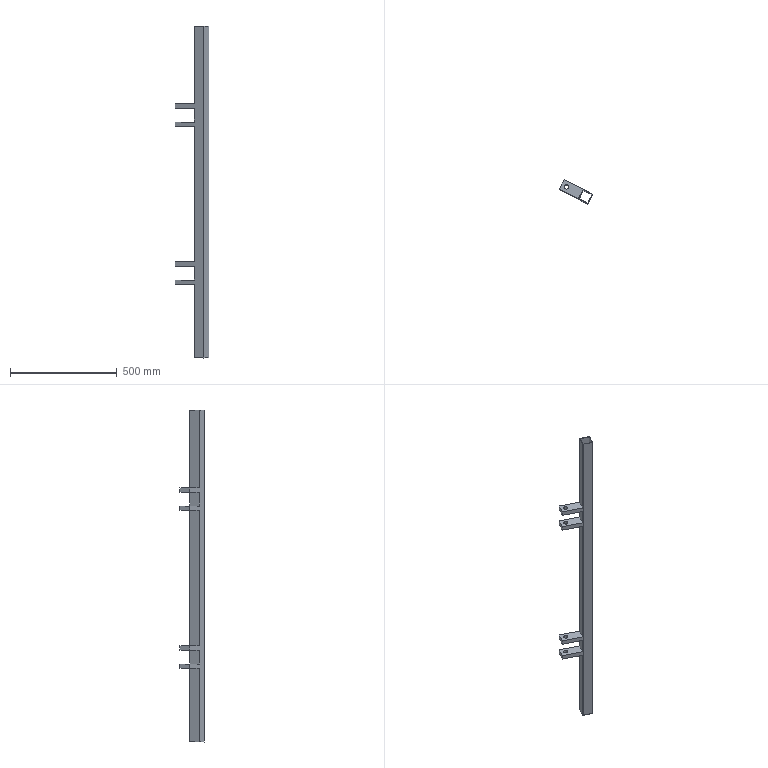Component | SolidWorks | Part13-1 | 1 solid | 34 faces | box 156.4 x 112.41 x 1554 mm | volume 971603 mm3 | plane 26 | cylinder 8 | commonest cylinder face diameters 20 x8
build123d program:
from build123d import *

# Parameters (mm, degrees)
SKETCH1_W           = 1554
SKETCH1_H           = 50
BOSS_EXTRUDE2_DEPTH = 50
SHELL1_T            = -2
SKETCH2_W           = 20
SKETCH2_H           = 100
BOSS_EXTRUDE3_DEPTH = 50
SKETCH3_R           = 10
CUT_EXTRUDE1_DEPTH  = 1195.898


with BuildPart() as part:
    # Sketch1 → Boss-Extrude2 (new body)
    with BuildSketch(Plane.XY):
        with Locations((715.859, 38.721)):
            Rectangle(SKETCH1_W, SKETCH1_H)
    extrude(amount=BOSS_EXTRUDE2_DEPTH)

    # Shell1
    shell1_openings = [part.faces().sort_by_distance(p)[0] for p in [
        (1492.859, 38.721, 25),
        (-61.141, 38.721, 25),
    ]]
    offset(amount=SHELL1_T, openings=shell1_openings, kind=Kind.INTERSECTION)

    # Sketch2 → Boss-Extrude3 (add)
    with BuildSketch(Plane.XZ.offset(-13.721)):
        with Locations((398.859, -50)):
            Rectangle(SKETCH2_W, SKETCH2_H)
        with Locations((313.859, -50)):
            Rectangle(SKETCH2_W, SKETCH2_H)
        with Locations((1052.859, -50)):
            Rectangle(SKETCH2_W, SKETCH2_H)
        with Locations((1137.859, -50)):
            Rectangle(SKETCH2_W, SKETCH2_H)
    extrude(amount=-BOSS_EXTRUDE3_DEPTH)

    # Sketch3 → Cut-Extrude1 (cut, through all)
    with BuildSketch(Plane.ZY.offset(-303.859)):
        with Locations((-75, 38.721)):
            Circle(SKETCH3_R)
    extrude(amount=-CUT_EXTRUDE1_DEPTH, mode=Mode.SUBTRACT)


solid = part.part

# Placed as in the assembly
solid = solid.moved(Location((-204.696, -928.158, 2528.83), (90, 63.121, -90)))
STEP:
#1=COLOUR_RGB('',0.7922,0.8196,0.9333);
#2=FILL_AREA_STYLE_COLOUR('',#1);
#3=FILL_AREA_STYLE('',(#2));
#4=SURFACE_STYLE_FILL_AREA(#3);
#5=SURFACE_SIDE_STYLE('',(#4));
#6=SURFACE_STYLE_USAGE(.BOTH.,#5);
#7=PRESENTATION_STYLE_ASSIGNMENT((#6));
#8=CARTESIAN_POINT('',(-9.652,-34.025,83.463));
#9=VERTEX_POINT('',#8);
#10=CARTESIAN_POINT('',(-10.355,-33.669,83.463));
#11=VERTEX_POINT('',#10);
#12=CARTESIAN_POINT('',(-10.003,-33.847,83.463));
#13=DIRECTION('',(0.,0.,-1.));
#14=DIRECTION('',(-0.892,0.4521,0.));
#15=AXIS2_PLACEMENT_3D('',#12,#13,#14);
#16=CIRCLE('',#15,0.3937);
#17=EDGE_CURVE('',#9,#11,#16,.T.);
#18=ORIENTED_EDGE('',*,*,#17,.T.);
#19=CARTESIAN_POINT('',(-10.355,-33.669,84.251));
#20=VERTEX_POINT('',#19);
#21=CARTESIAN_POINT('',(-10.355,-33.669,40.786));
#22=DIRECTION('',(-0.,-0.,1.));
#23=VECTOR('',#22,39.37);
#24=LINE('',#21,#23);
#25=EDGE_CURVE('',#11,#20,#24,.T.);
#26=ORIENTED_EDGE('',*,*,#25,.T.);
#27=CARTESIAN_POINT('',(-9.652,-34.025,84.251));
#28=VERTEX_POINT('',#27);
#29=CARTESIAN_POINT('',(-10.003,-33.847,84.251));
#30=DIRECTION('',(-0.,-0.,1.));
#31=DIRECTION('',(0.892,-0.4521,-0.));
#32=AXIS2_PLACEMENT_3D('',#29,#30,#31);
#33=CIRCLE('',#32,0.3937);
#34=EDGE_CURVE('',#20,#28,#33,.T.);
#35=ORIENTED_EDGE('',*,*,#34,.T.);
#36=CARTESIAN_POINT('',(-9.652,-34.025,40.786));
#37=DIRECTION('',(-0.,-0.,1.));
#38=VECTOR('',#37,39.37);
#39=LINE('',#36,#38);
#40=EDGE_CURVE('',#9,#28,#39,.T.);
#41=ORIENTED_EDGE('',*,*,#40,.F.);
#42=EDGE_LOOP('',(#18,#26,#35,#41));
#43=FACE_OUTER_BOUND('',#42,.T.);
#44=CARTESIAN_POINT('',(-10.003,-33.847,40.786));
#45=DIRECTION('',(-0.,-0.,1.));
#46=DIRECTION('',(0.892,-0.4521,-0.));
#47=AXIS2_PLACEMENT_3D('',#44,#45,#46);
#48=CYLINDRICAL_SURFACE('',#47,0.3937);
#49=ADVANCED_FACE('',(#43),#48,.F.);
#50=CARTESIAN_POINT('',(-9.652,-34.025,86.81));
#51=VERTEX_POINT('',#50);
#52=CARTESIAN_POINT('',(-10.355,-33.669,86.81));
#53=VERTEX_POINT('',#52);
#54=CARTESIAN_POINT('',(-10.003,-33.847,86.81));
#55=DIRECTION('',(0.,0.,-1.));
#56=DIRECTION('',(-0.892,0.4521,0.));
#57=AXIS2_PLACEMENT_3D('',#54,#55,#56);
#58=CIRCLE('',#57,0.3937);
#59=EDGE_CURVE('',#51,#53,#58,.T.);
#60=ORIENTED_EDGE('',*,*,#59,.T.);
#61=CARTESIAN_POINT('',(-10.355,-33.669,87.597));
#62=VERTEX_POINT('',#61);
#63=CARTESIAN_POINT('',(-10.355,-33.669,40.786));
#64=DIRECTION('',(-0.,-0.,1.));
#65=VECTOR('',#64,39.37);
#66=LINE('',#63,#65);
#67=EDGE_CURVE('',#53,#62,#66,.T.);
#68=ORIENTED_EDGE('',*,*,#67,.T.);
#69=CARTESIAN_POINT('',(-9.652,-34.025,87.597));
#70=VERTEX_POINT('',#69);
#71=CARTESIAN_POINT('',(-10.003,-33.847,87.597));
#72=DIRECTION('',(-0.,-0.,1.));
#73=DIRECTION('',(0.892,-0.4521,-0.));
#74=AXIS2_PLACEMENT_3D('',#71,#72,#73);
#75=CIRCLE('',#74,0.3937);
#76=EDGE_CURVE('',#62,#70,#75,.T.);
#77=ORIENTED_EDGE('',*,*,#76,.T.);
#78=CARTESIAN_POINT('',(-9.652,-34.025,40.786));
#79=DIRECTION('',(-0.,-0.,1.));
#80=VECTOR('',#79,39.37);
#81=LINE('',#78,#80);
#82=EDGE_CURVE('',#51,#70,#81,.T.);
#83=ORIENTED_EDGE('',*,*,#82,.F.);
#84=EDGE_LOOP('',(#60,#68,#77,#83));
#85=FACE_OUTER_BOUND('',#84,.T.);
#86=CARTESIAN_POINT('',(-10.003,-33.847,40.786));
#87=DIRECTION('',(-0.,-0.,1.));
#88=DIRECTION('',(0.892,-0.4521,-0.));
#89=AXIS2_PLACEMENT_3D('',#86,#87,#88);
#90=CYLINDRICAL_SURFACE('',#89,0.3937);
#91=ADVANCED_FACE('',(#85),#90,.F.);
#92=CARTESIAN_POINT('',(-9.652,-34.025,57.715));
#93=VERTEX_POINT('',#92);
#94=CARTESIAN_POINT('',(-10.355,-33.669,57.715));
#95=VERTEX_POINT('',#94);
#96=CARTESIAN_POINT('',(-10.003,-33.847,57.715));
#97=DIRECTION('',(0.,0.,-1.));
#98=DIRECTION('',(-0.892,0.4521,0.));
#99=AXIS2_PLACEMENT_3D('',#96,#97,#98);
#100=CIRCLE('',#99,0.3937);
#101=EDGE_CURVE('',#93,#95,#100,.T.);
#102=ORIENTED_EDGE('',*,*,#101,.T.);
#103=CARTESIAN_POINT('',(-10.355,-33.669,58.503));
#104=VERTEX_POINT('',#103);
#105=CARTESIAN_POINT('',(-10.355,-33.669,40.786));
#106=DIRECTION('',(-0.,-0.,1.));
#107=VECTOR('',#106,39.37);
#108=LINE('',#105,#107);
#109=EDGE_CURVE('',#95,#104,#108,.T.);
#110=ORIENTED_EDGE('',*,*,#109,.T.);
#111=CARTESIAN_POINT('',(-9.652,-34.025,58.503));
#112=VERTEX_POINT('',#111);
#113=CARTESIAN_POINT('',(-10.003,-33.847,58.503));
#114=DIRECTION('',(-0.,-0.,1.));
#115=DIRECTION('',(0.892,-0.4521,-0.));
#116=AXIS2_PLACEMENT_3D('',#113,#114,#115);
#117=CIRCLE('',#116,0.3937);
#118=EDGE_CURVE('',#104,#112,#117,.T.);
#119=ORIENTED_EDGE('',*,*,#118,.T.);
#120=CARTESIAN_POINT('',(-9.652,-34.025,40.786));
#121=DIRECTION('',(-0.,-0.,1.));
#122=VECTOR('',#121,39.37);
#123=LINE('',#120,#122);
#124=EDGE_CURVE('',#93,#112,#123,.T.);
#125=ORIENTED_EDGE('',*,*,#124,.F.);
#126=EDGE_LOOP('',(#102,#110,#119,#125));
#127=FACE_OUTER_BOUND('',#126,.T.);
#128=CARTESIAN_POINT('',(-10.003,-33.847,40.786));
#129=DIRECTION('',(-0.,-0.,1.));
#130=DIRECTION('',(0.892,-0.4521,-0.));
#131=AXIS2_PLACEMENT_3D('',#128,#129,#130);
#132=CYLINDRICAL_SURFACE('',#131,0.3937);
#133=ADVANCED_FACE('',(#127),#132,.F.);
#134=CARTESIAN_POINT('',(-9.652,-34.025,54.369));
#135=VERTEX_POINT('',#134);
#136=CARTESIAN_POINT('',(-10.355,-33.669,54.369));
#137=VERTEX_POINT('',#136);
#138=CARTESIAN_POINT('',(-10.003,-33.847,54.369));
#139=DIRECTION('',(0.,0.,-1.));
#140=DIRECTION('',(-0.892,0.4521,0.));
#141=AXIS2_PLACEMENT_3D('',#138,#139,#140);
#142=CIRCLE('',#141,0.3937);
#143=EDGE_CURVE('',#135,#137,#142,.T.);
#144=ORIENTED_EDGE('',*,*,#143,.T.);
#145=CARTESIAN_POINT('',(-10.355,-33.669,55.156));
#146=VERTEX_POINT('',#145);
#147=CARTESIAN_POINT('',(-10.355,-33.669,40.786));
#148=DIRECTION('',(-0.,-0.,1.));
#149=VECTOR('',#148,39.37);
#150=LINE('',#147,#149);
#151=EDGE_CURVE('',#137,#146,#150,.T.);
#152=ORIENTED_EDGE('',*,*,#151,.T.);
#153=CARTESIAN_POINT('',(-9.652,-34.025,55.156));
#154=VERTEX_POINT('',#153);
#155=CARTESIAN_POINT('',(-10.003,-33.847,55.156));
#156=DIRECTION('',(-0.,-0.,1.));
#157=DIRECTION('',(0.892,-0.4521,-0.));
#158=AXIS2_PLACEMENT_3D('',#155,#156,#157);
#159=CIRCLE('',#158,0.3937);
#160=EDGE_CURVE('',#146,#154,#159,.T.);
#161=ORIENTED_EDGE('',*,*,#160,.T.);
#162=CARTESIAN_POINT('',(-9.652,-34.025,40.786));
#163=DIRECTION('',(-0.,-0.,1.));
#164=VECTOR('',#163,39.37);
#165=LINE('',#162,#164);
#166=EDGE_CURVE('',#135,#154,#165,.T.);
#167=ORIENTED_EDGE('',*,*,#166,.F.);
#168=EDGE_LOOP('',(#144,#152,#161,#167));
#169=FACE_OUTER_BOUND('',#168,.T.);
#170=CARTESIAN_POINT('',(-10.003,-33.847,40.786));
#171=DIRECTION('',(-0.,-0.,1.));
#172=DIRECTION('',(0.892,-0.4521,-0.));
#173=AXIS2_PLACEMENT_3D('',#170,#171,#172);
#174=CYLINDRICAL_SURFACE('',#173,0.3937);
#175=ADVANCED_FACE('',(#169),#174,.F.);
#176=CARTESIAN_POINT('',(-6.925,-34.304,54.369));
#177=VERTEX_POINT('',#176);
#178=CARTESIAN_POINT('',(-7.815,-36.06,54.369));
#179=VERTEX_POINT('',#178);
#180=CARTESIAN_POINT('',(-6.925,-34.304,54.369));
#181=DIRECTION('',(-0.4521,-0.892,-0.));
#182=VECTOR('',#181,39.37);
#183=LINE('',#180,#182);
#184=EDGE_CURVE('',#177,#179,#183,.T.);
#185=ORIENTED_EDGE('',*,*,#184,.F.);
#186=CARTESIAN_POINT('',(-6.925,-34.304,40.786));
#187=VERTEX_POINT('',#186);
#188=CARTESIAN_POINT('',(-6.925,-34.304,101.967));
#189=DIRECTION('',(-0.,-0.,1.));
#190=VECTOR('',#189,39.37);
#191=LINE('',#188,#190);
#192=EDGE_CURVE('',#187,#177,#191,.T.);
#193=ORIENTED_EDGE('',*,*,#192,.F.);
#194=CARTESIAN_POINT('',(-7.815,-36.06,40.786));
#195=VERTEX_POINT('',#194);
#196=CARTESIAN_POINT('',(-6.925,-34.304,40.786));
#197=DIRECTION('',(0.4521,0.892,0.));
#198=VECTOR('',#197,39.37);
#199=LINE('',#196,#198);
#200=EDGE_CURVE('',#195,#187,#199,.T.);
#201=ORIENTED_EDGE('',*,*,#200,.F.);
#202=CARTESIAN_POINT('',(-7.815,-36.06,101.967));
#203=DIRECTION('',(0.,0.,-1.));
#204=VECTOR('',#203,39.37);
#205=LINE('',#202,#204);
#206=EDGE_CURVE('',#179,#195,#205,.T.);
#207=ORIENTED_EDGE('',*,*,#206,.F.);
#208=EDGE_LOOP('',(#185,#193,#201,#207));
#209=FACE_OUTER_BOUND('',#208,.T.);
#210=CARTESIAN_POINT('',(-8.059,-36.542,99.56));
#211=DIRECTION('',(0.892,-0.4521,-0.));
#212=DIRECTION('',(0.,0.,-1.));
#213=AXIS2_PLACEMENT_3D('',#210,#211,#212);
#214=PLANE('',#213);
#215=ADVANCED_FACE('',(#209),#214,.F.);
#216=CARTESIAN_POINT('',(-6.925,-34.304,55.156));
#217=VERTEX_POINT('',#216);
#218=CARTESIAN_POINT('',(-6.925,-34.304,57.715));
#219=VERTEX_POINT('',#218);
#220=CARTESIAN_POINT('',(-6.925,-34.304,101.967));
#221=DIRECTION('',(-0.,-0.,1.));
#222=VECTOR('',#221,39.37);
#223=LINE('',#220,#222);
#224=EDGE_CURVE('',#217,#219,#223,.T.);
#225=ORIENTED_EDGE('',*,*,#224,.F.);
#226=CARTESIAN_POINT('',(-7.815,-36.06,55.156));
#227=VERTEX_POINT('',#226);
#228=CARTESIAN_POINT('',(-6.925,-34.304,55.156));
#229=DIRECTION('',(-0.4521,-0.892,-0.));
#230=VECTOR('',#229,39.37);
#231=LINE('',#228,#230);
#232=EDGE_CURVE('',#217,#227,#231,.T.);
#233=ORIENTED_EDGE('',*,*,#232,.T.);
#234=CARTESIAN_POINT('',(-7.815,-36.06,57.715));
#235=VERTEX_POINT('',#234);
#236=CARTESIAN_POINT('',(-7.815,-36.06,101.967));
#237=DIRECTION('',(0.,0.,-1.));
#238=VECTOR('',#237,39.37);
#239=LINE('',#236,#238);
#240=EDGE_CURVE('',#235,#227,#239,.T.);
#241=ORIENTED_EDGE('',*,*,#240,.F.);
#242=CARTESIAN_POINT('',(-6.925,-34.304,57.715));
#243=DIRECTION('',(-0.4521,-0.892,-0.));
#244=VECTOR('',#243,39.37);
#245=LINE('',#242,#244);
#246=EDGE_CURVE('',#219,#235,#245,.T.);
#247=ORIENTED_EDGE('',*,*,#246,.F.);
#248=EDGE_LOOP('',(#225,#233,#241,#247));
#249=FACE_OUTER_BOUND('',#248,.T.);
#250=CARTESIAN_POINT('',(-8.059,-36.542,99.56));
#251=DIRECTION('',(0.892,-0.4521,-0.));
#252=DIRECTION('',(0.,0.,-1.));
#253=AXIS2_PLACEMENT_3D('',#250,#251,#252);
#254=PLANE('',#253);
#255=ADVANCED_FACE('',(#249),#254,.F.);
#256=CARTESIAN_POINT('',(-6.925,-34.304,86.81));
#257=VERTEX_POINT('',#256);
#258=CARTESIAN_POINT('',(-7.815,-36.06,86.81));
#259=VERTEX_POINT('',#258);
#260=CARTESIAN_POINT('',(-6.925,-34.304,86.81));
#261=DIRECTION('',(-0.4521,-0.892,-0.));
#262=VECTOR('',#261,39.37);
#263=LINE('',#260,#262);
#264=EDGE_CURVE('',#257,#259,#263,.T.);
#265=ORIENTED_EDGE('',*,*,#264,.F.);
#266=CARTESIAN_POINT('',(-6.925,-34.304,84.251));
#267=VERTEX_POINT('',#266);
#268=CARTESIAN_POINT('',(-6.925,-34.304,101.967));
#269=DIRECTION('',(-0.,-0.,1.));
#270=VECTOR('',#269,39.37);
#271=LINE('',#268,#270);
#272=EDGE_CURVE('',#267,#257,#271,.T.);
#273=ORIENTED_EDGE('',*,*,#272,.F.);
#274=CARTESIAN_POINT('',(-7.815,-36.06,84.251));
#275=VERTEX_POINT('',#274);
#276=CARTESIAN_POINT('',(-6.925,-34.304,84.251));
#277=DIRECTION('',(-0.4521,-0.892,-0.));
#278=VECTOR('',#277,39.37);
#279=LINE('',#276,#278);
#280=EDGE_CURVE('',#267,#275,#279,.T.);
#281=ORIENTED_EDGE('',*,*,#280,.T.);
#282=CARTESIAN_POINT('',(-7.815,-36.06,101.967));
#283=DIRECTION('',(0.,0.,-1.));
#284=VECTOR('',#283,39.37);
#285=LINE('',#282,#284);
#286=EDGE_CURVE('',#259,#275,#285,.T.);
#287=ORIENTED_EDGE('',*,*,#286,.F.);
#288=EDGE_LOOP('',(#265,#273,#281,#287));
#289=FACE_OUTER_BOUND('',#288,.T.);
#290=CARTESIAN_POINT('',(-8.059,-36.542,99.56));
#291=DIRECTION('',(0.892,-0.4521,-0.));
#292=DIRECTION('',(0.,0.,-1.));
#293=AXIS2_PLACEMENT_3D('',#290,#291,#292);
#294=PLANE('',#293);
#295=ADVANCED_FACE('',(#289),#294,.F.);
#296=CARTESIAN_POINT('',(-6.925,-34.304,58.503));
#297=VERTEX_POINT('',#296);
#298=CARTESIAN_POINT('',(-6.925,-34.304,83.463));
#299=VERTEX_POINT('',#298);
#300=CARTESIAN_POINT('',(-6.925,-34.304,101.967));
#301=DIRECTION('',(-0.,-0.,1.));
#302=VECTOR('',#301,39.37);
#303=LINE('',#300,#302);
#304=EDGE_CURVE('',#297,#299,#303,.T.);
#305=ORIENTED_EDGE('',*,*,#304,.F.);
#306=CARTESIAN_POINT('',(-7.815,-36.06,58.503));
#307=VERTEX_POINT('',#306);
#308=CARTESIAN_POINT('',(-6.925,-34.304,58.503));
#309=DIRECTION('',(-0.4521,-0.892,-0.));
#310=VECTOR('',#309,39.37);
#311=LINE('',#308,#310);
#312=EDGE_CURVE('',#297,#307,#311,.T.);
#313=ORIENTED_EDGE('',*,*,#312,.T.);
#314=CARTESIAN_POINT('',(-7.815,-36.06,83.463));
#315=VERTEX_POINT('',#314);
#316=CARTESIAN_POINT('',(-7.815,-36.06,101.967));
#317=DIRECTION('',(0.,0.,-1.));
#318=VECTOR('',#317,39.37);
#319=LINE('',#316,#318);
#320=EDGE_CURVE('',#315,#307,#319,.T.);
#321=ORIENTED_EDGE('',*,*,#320,.F.);
#322=CARTESIAN_POINT('',(-6.925,-34.304,83.463));
#323=DIRECTION('',(-0.4521,-0.892,-0.));
#324=VECTOR('',#323,39.37);
#325=LINE('',#322,#324);
#326=EDGE_CURVE('',#299,#315,#325,.T.);
#327=ORIENTED_EDGE('',*,*,#326,.F.);
#328=EDGE_LOOP('',(#305,#313,#321,#327));
#329=FACE_OUTER_BOUND('',#328,.T.);
#330=CARTESIAN_POINT('',(-8.059,-36.542,99.56));
#331=DIRECTION('',(0.892,-0.4521,-0.));
#332=DIRECTION('',(0.,0.,-1.));
#333=AXIS2_PLACEMENT_3D('',#330,#331,#332);
#334=PLANE('',#333);
#335=ADVANCED_FACE('',(#329),#334,.F.);
#336=CARTESIAN_POINT('',(-6.925,-34.304,101.967));
#337=VERTEX_POINT('',#336);
#338=CARTESIAN_POINT('',(-7.815,-36.06,101.967));
#339=VERTEX_POINT('',#338);
#340=CARTESIAN_POINT('',(-6.925,-34.304,101.967));
#341=DIRECTION('',(-0.4521,-0.892,-0.));
#342=VECTOR('',#341,39.37);
#343=LINE('',#340,#342);
#344=EDGE_CURVE('',#337,#339,#343,.T.);
#345=ORIENTED_EDGE('',*,*,#344,.T.);
#346=CARTESIAN_POINT('',(-6.059,-36.95,101.967));
#347=VERTEX_POINT('',#346);
#348=CARTESIAN_POINT('',(-6.059,-36.95,101.967));
#349=DIRECTION('',(-0.892,0.4521,0.));
#350=VECTOR('',#349,39.37);
#351=LINE('',#348,#350);
#352=EDGE_CURVE('',#347,#339,#351,.T.);
#353=ORIENTED_EDGE('',*,*,#352,.F.);
#354=CARTESIAN_POINT('',(-5.169,-35.194,101.967));
#355=VERTEX_POINT('',#354);
#356=CARTESIAN_POINT('',(-5.169,-35.194,101.967));
#357=DIRECTION('',(-0.4521,-0.892,-0.));
#358=VECTOR('',#357,39.37);
#359=LINE('',#356,#358);
#360=EDGE_CURVE('',#355,#347,#359,.T.);
#361=ORIENTED_EDGE('',*,*,#360,.F.);
#362=CARTESIAN_POINT('',(-5.169,-35.194,101.967));
#363=DIRECTION('',(-0.892,0.4521,0.));
#364=VECTOR('',#363,39.37);
#365=LINE('',#362,#364);
#366=EDGE_CURVE('',#355,#337,#365,.T.);
#367=ORIENTED_EDGE('',*,*,#366,.T.);
#368=EDGE_LOOP('',(#345,#353,#361,#367));
#369=FACE_OUTER_BOUND('',#368,.T.);
#370=CARTESIAN_POINT('',(-6.89,-34.41,101.967));
#371=VERTEX_POINT('',#370);
#372=CARTESIAN_POINT('',(-7.709,-36.025,101.967));
#373=VERTEX_POINT('',#372);
#374=CARTESIAN_POINT('',(-6.854,-34.34,101.967));
#375=DIRECTION('',(-0.4521,-0.892,-0.));
#376=VECTOR('',#375,39.37);
#377=LINE('',#374,#376);
#378=EDGE_CURVE('',#371,#373,#377,.T.);
#379=ORIENTED_EDGE('',*,*,#378,.F.);
#380=CARTESIAN_POINT('',(-5.275,-35.229,101.967));
#381=VERTEX_POINT('',#380);
#382=CARTESIAN_POINT('',(-5.204,-35.264,101.967));
#383=DIRECTION('',(-0.892,0.4521,0.));
#384=VECTOR('',#383,39.37);
#385=LINE('',#382,#384);
#386=EDGE_CURVE('',#381,#371,#385,.T.);
#387=ORIENTED_EDGE('',*,*,#386,.F.);
#388=CARTESIAN_POINT('',(-6.093,-36.844,101.967));
#389=VERTEX_POINT('',#388);
#390=CARTESIAN_POINT('',(-5.239,-35.158,101.967));
#391=DIRECTION('',(-0.4521,-0.892,-0.));
#392=VECTOR('',#391,39.37);
#393=LINE('',#390,#392);
#394=EDGE_CURVE('',#381,#389,#393,.T.);
#395=ORIENTED_EDGE('',*,*,#394,.T.);
#396=CARTESIAN_POINT('',(-6.023,-36.88,101.967));
#397=DIRECTION('',(-0.892,0.4521,0.));
#398=VECTOR('',#397,39.37);
#399=LINE('',#396,#398);
#400=EDGE_CURVE('',#389,#373,#399,.T.);
#401=ORIENTED_EDGE('',*,*,#400,.T.);
#402=EDGE_LOOP('',(#379,#387,#395,#401));
#403=FACE_BOUND('',#402,.T.);
#404=CARTESIAN_POINT('',(-5.169,-35.194,101.967));
#405=DIRECTION('',(0.,0.,-1.));
#406=DIRECTION('',(0.4521,0.892,0.));
#407=AXIS2_PLACEMENT_3D('',#404,#405,#406);
#408=PLANE('',#407);
#409=ADVANCED_FACE('',(#369,#403),#408,.F.);
#410=ORIENTED_EDGE('',*,*,#200,.T.);
#411=CARTESIAN_POINT('',(-5.169,-35.194,40.786));
#412=VERTEX_POINT('',#411);
#413=CARTESIAN_POINT('',(-5.169,-35.194,40.786));
#414=DIRECTION('',(-0.892,0.4521,0.));
#415=VECTOR('',#414,39.37);
#416=LINE('',#413,#415);
#417=EDGE_CURVE('',#412,#187,#416,.T.);
#418=ORIENTED_EDGE('',*,*,#417,.F.);
#419=CARTESIAN_POINT('',(-6.059,-36.95,40.786));
#420=VERTEX_POINT('',#419);
#421=CARTESIAN_POINT('',(-5.169,-35.194,40.786));
#422=DIRECTION('',(0.4521,0.892,0.));
#423=VECTOR('',#422,39.37);
#424=LINE('',#421,#423);
#425=EDGE_CURVE('',#420,#412,#424,.T.);
#426=ORIENTED_EDGE('',*,*,#425,.F.);
#427=CARTESIAN_POINT('',(-6.059,-36.95,40.786));
#428=DIRECTION('',(-0.892,0.4521,0.));
#429=VECTOR('',#428,39.37);
#430=LINE('',#427,#429);
#431=EDGE_CURVE('',#420,#195,#430,.T.);
#432=ORIENTED_EDGE('',*,*,#431,.T.);
#433=EDGE_LOOP('',(#410,#418,#426,#432));
#434=FACE_OUTER_BOUND('',#433,.T.);
#435=CARTESIAN_POINT('',(-7.709,-36.025,40.786));
#436=VERTEX_POINT('',#435);
#437=CARTESIAN_POINT('',(-6.89,-34.41,40.786));
#438=VERTEX_POINT('',#437);
#439=CARTESIAN_POINT('',(-6.854,-34.34,40.786));
#440=DIRECTION('',(0.4521,0.892,0.));
#441=VECTOR('',#440,39.37);
#442=LINE('',#439,#441);
#443=EDGE_CURVE('',#436,#438,#442,.T.);
#444=ORIENTED_EDGE('',*,*,#443,.F.);
#445=CARTESIAN_POINT('',(-6.093,-36.844,40.786));
#446=VERTEX_POINT('',#445);
#447=CARTESIAN_POINT('',(-6.023,-36.88,40.786));
#448=DIRECTION('',(-0.892,0.4521,0.));
#449=VECTOR('',#448,39.37);
#450=LINE('',#447,#449);
#451=EDGE_CURVE('',#446,#436,#450,.T.);
#452=ORIENTED_EDGE('',*,*,#451,.F.);
#453=CARTESIAN_POINT('',(-5.275,-35.229,40.786));
#454=VERTEX_POINT('',#453);
#455=CARTESIAN_POINT('',(-5.239,-35.158,40.786));
#456=DIRECTION('',(0.4521,0.892,0.));
#457=VECTOR('',#456,39.37);
#458=LINE('',#455,#457);
#459=EDGE_CURVE('',#446,#454,#458,.T.);
#460=ORIENTED_EDGE('',*,*,#459,.T.);
#461=CARTESIAN_POINT('',(-5.204,-35.264,40.786));
#462=DIRECTION('',(-0.892,0.4521,0.));
#463=VECTOR('',#462,39.37);
#464=LINE('',#461,#463);
#465=EDGE_CURVE('',#454,#438,#464,.T.);
#466=ORIENTED_EDGE('',*,*,#465,.T.);
#467=EDGE_LOOP('',(#444,#452,#460,#466));
#468=FACE_BOUND('',#467,.T.);
#469=CARTESIAN_POINT('',(-5.169,-35.194,40.786));
#470=DIRECTION('',(-0.,-0.,1.));
#471=DIRECTION('',(0.892,-0.4521,-0.));
#472=AXIS2_PLACEMENT_3D('',#469,#470,#471);
#473=PLANE('',#472);
#474=ADVANCED_FACE('',(#434,#468),#473,.F.);
#475=CARTESIAN_POINT('',(-7.815,-36.06,87.597));
#476=VERTEX_POINT('',#475);
#477=CARTESIAN_POINT('',(-7.815,-36.06,101.967));
#478=DIRECTION('',(0.,0.,-1.));
#479=VECTOR('',#478,39.37);
#480=LINE('',#477,#479);
#481=EDGE_CURVE('',#339,#476,#480,.T.);
#482=ORIENTED_EDGE('',*,*,#481,.T.);
#483=CARTESIAN_POINT('',(-11.326,-34.28,87.597));
#484=VERTEX_POINT('',#483);
#485=CARTESIAN_POINT('',(-7.815,-36.06,87.597));
#486=DIRECTION('',(-0.892,0.4521,0.));
#487=VECTOR('',#486,39.37);
#488=LINE('',#485,#487);
#489=EDGE_CURVE('',#476,#484,#488,.T.);
#490=ORIENTED_EDGE('',*,*,#489,.T.);
#491=CARTESIAN_POINT('',(-11.326,-34.28,86.81));
#492=VERTEX_POINT('',#491);
#493=CARTESIAN_POINT('',(-11.326,-34.28,86.81));
#494=DIRECTION('',(0.,0.,-1.));
#495=VECTOR('',#494,39.37);
#496=LINE('',#493,#495);
#497=EDGE_CURVE('',#484,#492,#496,.T.);
#498=ORIENTED_EDGE('',*,*,#497,.T.);
#499=CARTESIAN_POINT('',(-7.815,-36.06,86.81));
#500=DIRECTION('',(0.892,-0.4521,-0.));
#501=VECTOR('',#500,39.37);
#502=LINE('',#499,#501);
#503=EDGE_CURVE('',#492,#259,#502,.T.);
#504=ORIENTED_EDGE('',*,*,#503,.T.);
#505=ORIENTED_EDGE('',*,*,#286,.T.);
#506=CARTESIAN_POINT('',(-11.326,-34.28,84.251));
#507=VERTEX_POINT('',#506);
#508=CARTESIAN_POINT('',(-7.815,-36.06,84.251));
#509=DIRECTION('',(-0.892,0.4521,0.));
#510=VECTOR('',#509,39.37);
#511=LINE('',#508,#510);
#512=EDGE_CURVE('',#275,#507,#511,.T.);
#513=ORIENTED_EDGE('',*,*,#512,.T.);
#514=CARTESIAN_POINT('',(-11.326,-34.28,83.463));
#515=VERTEX_POINT('',#514);
#516=CARTESIAN_POINT('',(-11.326,-34.28,84.251));
#517=DIRECTION('',(0.,0.,-1.));
#518=VECTOR('',#517,39.37);
#519=LINE('',#516,#518);
#520=EDGE_CURVE('',#507,#515,#519,.T.);
#521=ORIENTED_EDGE('',*,*,#520,.T.);
#522=CARTESIAN_POINT('',(-7.815,-36.06,83.463));
#523=DIRECTION('',(0.892,-0.4521,-0.));
#524=VECTOR('',#523,39.37);
#525=LINE('',#522,#524);
#526=EDGE_CURVE('',#515,#315,#525,.T.);
#527=ORIENTED_EDGE('',*,*,#526,.T.);
#528=ORIENTED_EDGE('',*,*,#320,.T.);
#529=CARTESIAN_POINT('',(-11.326,-34.28,58.503));
#530=VERTEX_POINT('',#529);
#531=CARTESIAN_POINT('',(-7.815,-36.06,58.503));
#532=DIRECTION('',(-0.892,0.4521,0.));
#533=VECTOR('',#532,39.37);
#534=LINE('',#531,#533);
#535=EDGE_CURVE('',#307,#530,#534,.T.);
#536=ORIENTED_EDGE('',*,*,#535,.T.);
#537=CARTESIAN_POINT('',(-11.326,-34.28,57.715));
#538=VERTEX_POINT('',#537);
#539=CARTESIAN_POINT('',(-11.326,-34.28,57.715));
#540=DIRECTION('',(0.,0.,-1.));
#541=VECTOR('',#540,39.37);
#542=LINE('',#539,#541);
#543=EDGE_CURVE('',#530,#538,#542,.T.);
#544=ORIENTED_EDGE('',*,*,#543,.T.);
#545=CARTESIAN_POINT('',(-7.815,-36.06,57.715));
#546=DIRECTION('',(0.892,-0.4521,-0.));
#547=VECTOR('',#546,39.37);
#548=LINE('',#545,#547);
#549=EDGE_CURVE('',#538,#235,#548,.T.);
#550=ORIENTED_EDGE('',*,*,#549,.T.);
#551=ORIENTED_EDGE('',*,*,#240,.T.);
#552=CARTESIAN_POINT('',(-11.326,-34.28,55.156));
#553=VERTEX_POINT('',#552);
#554=CARTESIAN_POINT('',(-7.815,-36.06,55.156));
#555=DIRECTION('',(-0.892,0.4521,0.));
#556=VECTOR('',#555,39.37);
#557=LINE('',#554,#556);
#558=EDGE_CURVE('',#227,#553,#557,.T.);
#559=ORIENTED_EDGE('',*,*,#558,.T.);
#560=CARTESIAN_POINT('',(-11.326,-34.28,54.369));
#561=VERTEX_POINT('',#560);
#562=CARTESIAN_POINT('',(-11.326,-34.28,55.156));
#563=DIRECTION('',(0.,0.,-1.));
#564=VECTOR('',#563,39.37);
#565=LINE('',#562,#564);
#566=EDGE_CURVE('',#553,#561,#565,.T.);
#567=ORIENTED_EDGE('',*,*,#566,.T.);
#568=CARTESIAN_POINT('',(-7.815,-36.06,54.369));
#569=DIRECTION('',(0.892,-0.4521,-0.));
#570=VECTOR('',#569,39.37);
#571=LINE('',#568,#570);
#572=EDGE_CURVE('',#561,#179,#571,.T.);
#573=ORIENTED_EDGE('',*,*,#572,.T.);
#574=ORIENTED_EDGE('',*,*,#206,.T.);
#575=ORIENTED_EDGE('',*,*,#431,.F.);
#576=CARTESIAN_POINT('',(-6.059,-36.95,101.967));
#577=DIRECTION('',(0.,0.,-1.));
#578=VECTOR('',#577,39.37);
#579=LINE('',#576,#578);
#580=EDGE_CURVE('',#347,#420,#579,.T.);
#581=ORIENTED_EDGE('',*,*,#580,.F.);
#582=ORIENTED_EDGE('',*,*,#352,.T.);
#583=EDGE_LOOP('',(#482,#490,#498,#504,#505,#513,#521,#527,#528,#536,#544,#550,#551,#559,#567,#573,#574,#575,#581,#582));
#584=FACE_OUTER_BOUND('',#583,.T.);
#585=CARTESIAN_POINT('',(-6.059,-36.95,101.967));
#586=DIRECTION('',(0.4521,0.892,0.));
#587=DIRECTION('',(0.892,-0.4521,-0.));
#588=AXIS2_PLACEMENT_3D('',#585,#586,#587);
#589=PLANE('',#588);
#590=ADVANCED_FACE('',(#584),#589,.F.);
#591=ORIENTED_EDGE('',*,*,#192,.T.);
#592=CARTESIAN_POINT('',(-10.436,-32.524,54.369));
#593=VERTEX_POINT('',#592);
#594=CARTESIAN_POINT('',(-6.925,-34.304,54.369));
#595=DIRECTION('',(0.892,-0.4521,-0.));
#596=VECTOR('',#595,39.37);
#597=LINE('',#594,#596);
#598=EDGE_CURVE('',#593,#177,#597,.T.);
#599=ORIENTED_EDGE('',*,*,#598,.F.);
#600=CARTESIAN_POINT('',(-10.436,-32.524,55.156));
#601=VERTEX_POINT('',#600);
#602=CARTESIAN_POINT('',(-10.436,-32.524,55.156));
#603=DIRECTION('',(0.,0.,-1.));
#604=VECTOR('',#603,39.37);
#605=LINE('',#602,#604);
#606=EDGE_CURVE('',#601,#593,#605,.T.);
#607=ORIENTED_EDGE('',*,*,#606,.F.);
#608=CARTESIAN_POINT('',(-6.925,-34.304,55.156));
#609=DIRECTION('',(-0.892,0.4521,0.));
#610=VECTOR('',#609,39.37);
#611=LINE('',#608,#610);
#612=EDGE_CURVE('',#217,#601,#611,.T.);
#613=ORIENTED_EDGE('',*,*,#612,.F.);
#614=ORIENTED_EDGE('',*,*,#224,.T.);
#615=CARTESIAN_POINT('',(-10.436,-32.524,57.715));
#616=VERTEX_POINT('',#615);
#617=CARTESIAN_POINT('',(-6.925,-34.304,57.715));
#618=DIRECTION('',(0.892,-0.4521,-0.));
#619=VECTOR('',#618,39.37);
#620=LINE('',#617,#619);
#621=EDGE_CURVE('',#616,#219,#620,.T.);
#622=ORIENTED_EDGE('',*,*,#621,.F.);
#623=CARTESIAN_POINT('',(-10.436,-32.524,58.503));
#624=VERTEX_POINT('',#623);
#625=CARTESIAN_POINT('',(-10.436,-32.524,57.715));
#626=DIRECTION('',(0.,0.,-1.));
#627=VECTOR('',#626,39.37);
#628=LINE('',#625,#627);
#629=EDGE_CURVE('',#624,#616,#628,.T.);
#630=ORIENTED_EDGE('',*,*,#629,.F.);
#631=CARTESIAN_POINT('',(-6.925,-34.304,58.503));
#632=DIRECTION('',(-0.892,0.4521,0.));
#633=VECTOR('',#632,39.37);
#634=LINE('',#631,#633);
#635=EDGE_CURVE('',#297,#624,#634,.T.);
#636=ORIENTED_EDGE('',*,*,#635,.F.);
#637=ORIENTED_EDGE('',*,*,#304,.T.);
#638=CARTESIAN_POINT('',(-10.436,-32.524,83.463));
#639=VERTEX_POINT('',#638);
#640=CARTESIAN_POINT('',(-6.925,-34.304,83.463));
#641=DIRECTION('',(0.892,-0.4521,-0.));
#642=VECTOR('',#641,39.37);
#643=LINE('',#640,#642);
#644=EDGE_CURVE('',#639,#299,#643,.T.);
#645=ORIENTED_EDGE('',*,*,#644,.F.);
#646=CARTESIAN_POINT('',(-10.436,-32.524,84.251));
#647=VERTEX_POINT('',#646);
#648=CARTESIAN_POINT('',(-10.436,-32.524,84.251));
#649=DIRECTION('',(0.,0.,-1.));
#650=VECTOR('',#649,39.37);
#651=LINE('',#648,#650);
#652=EDGE_CURVE('',#647,#639,#651,.T.);
#653=ORIENTED_EDGE('',*,*,#652,.F.);
#654=CARTESIAN_POINT('',(-6.925,-34.304,84.251));
#655=DIRECTION('',(-0.892,0.4521,0.));
#656=VECTOR('',#655,39.37);
#657=LINE('',#654,#656);
#658=EDGE_CURVE('',#267,#647,#657,.T.);
#659=ORIENTED_EDGE('',*,*,#658,.F.);
#660=ORIENTED_EDGE('',*,*,#272,.T.);
#661=CARTESIAN_POINT('',(-10.436,-32.524,86.81));
#662=VERTEX_POINT('',#661);
#663=CARTESIAN_POINT('',(-6.925,-34.304,86.81));
#664=DIRECTION('',(0.892,-0.4521,-0.));
#665=VECTOR('',#664,39.37);
#666=LINE('',#663,#665);
#667=EDGE_CURVE('',#662,#257,#666,.T.);
#668=ORIENTED_EDGE('',*,*,#667,.F.);
#669=CARTESIAN_POINT('',(-10.436,-32.524,87.597));
#670=VERTEX_POINT('',#669);
#671=CARTESIAN_POINT('',(-10.436,-32.524,86.81));
#672=DIRECTION('',(0.,0.,-1.));
#673=VECTOR('',#672,39.37);
#674=LINE('',#671,#673);
#675=EDGE_CURVE('',#670,#662,#674,.T.);
#676=ORIENTED_EDGE('',*,*,#675,.F.);
#677=CARTESIAN_POINT('',(-6.925,-34.304,87.597));
#678=VERTEX_POINT('',#677);
#679=CARTESIAN_POINT('',(-6.925,-34.304,87.597));
#680=DIRECTION('',(-0.892,0.4521,0.));
#681=VECTOR('',#680,39.37);
#682=LINE('',#679,#681);
#683=EDGE_CURVE('',#678,#670,#682,.T.);
#684=ORIENTED_EDGE('',*,*,#683,.F.);
#685=CARTESIAN_POINT('',(-6.925,-34.304,101.967));
#686=DIRECTION('',(-0.,-0.,1.));
#687=VECTOR('',#686,39.37);
#688=LINE('',#685,#687);
#689=EDGE_CURVE('',#678,#337,#688,.T.);
#690=ORIENTED_EDGE('',*,*,#689,.T.);
#691=ORIENTED_EDGE('',*,*,#366,.F.);
#692=CARTESIAN_POINT('',(-5.169,-35.194,101.967));
#693=DIRECTION('',(-0.,-0.,1.));
#694=VECTOR('',#693,39.37);
#695=LINE('',#692,#694);
#696=EDGE_CURVE('',#412,#355,#695,.T.);
#697=ORIENTED_EDGE('',*,*,#696,.F.);
#698=ORIENTED_EDGE('',*,*,#417,.T.);
#699=EDGE_LOOP('',(#591,#599,#607,#613,#614,#622,#630,#636,#637,#645,#653,#659,#660,#668,#676,#684,#690,#691,#697,#698));
#700=FACE_OUTER_BOUND('',#699,.T.);
#701=CARTESIAN_POINT('',(-5.169,-35.194,101.967));
#702=DIRECTION('',(-0.4521,-0.892,-0.));
#703=DIRECTION('',(-0.892,0.4521,0.));
#704=AXIS2_PLACEMENT_3D('',#701,#702,#703);
#705=PLANE('',#704);
#706=ADVANCED_FACE('',(#700),#705,.F.);
#707=ORIENTED_EDGE('',*,*,#360,.T.);
#708=ORIENTED_EDGE('',*,*,#580,.T.);
#709=ORIENTED_EDGE('',*,*,#425,.T.);
#710=ORIENTED_EDGE('',*,*,#696,.T.);
#711=EDGE_LOOP('',(#707,#708,#709,#710));
#712=FACE_OUTER_BOUND('',#711,.T.);
#713=CARTESIAN_POINT('',(-6.303,-37.432,99.56));
#714=DIRECTION('',(0.892,-0.4521,-0.));
#715=DIRECTION('',(0.,0.,-1.));
#716=AXIS2_PLACEMENT_3D('',#713,#714,#715);
#717=PLANE('',#716);
#718=ADVANCED_FACE('',(#712),#717,.T.);
#719=ORIENTED_EDGE('',*,*,#689,.F.);
#720=CARTESIAN_POINT('',(-6.925,-34.304,87.597));
#721=DIRECTION('',(-0.4521,-0.892,-0.));
#722=VECTOR('',#721,39.37);
#723=LINE('',#720,#722);
#724=EDGE_CURVE('',#678,#476,#723,.T.);
#725=ORIENTED_EDGE('',*,*,#724,.T.);
#726=ORIENTED_EDGE('',*,*,#481,.F.);
#727=ORIENTED_EDGE('',*,*,#344,.F.);
#728=EDGE_LOOP('',(#719,#725,#726,#727));
#729=FACE_OUTER_BOUND('',#728,.T.);
#730=CARTESIAN_POINT('',(-8.059,-36.542,99.56));
#731=DIRECTION('',(0.892,-0.4521,-0.));
#732=DIRECTION('',(0.,0.,-1.));
#733=AXIS2_PLACEMENT_3D('',#730,#731,#732);
#734=PLANE('',#733);
#735=ADVANCED_FACE('',(#729),#734,.F.);
#736=CARTESIAN_POINT('',(-7.709,-36.025,101.967));
#737=DIRECTION('',(0.,0.,-1.));
#738=VECTOR('',#737,39.37);
#739=LINE('',#736,#738);
#740=EDGE_CURVE('',#373,#436,#739,.T.);
#741=ORIENTED_EDGE('',*,*,#740,.F.);
#742=ORIENTED_EDGE('',*,*,#400,.F.);
#743=CARTESIAN_POINT('',(-6.093,-36.844,101.967));
#744=DIRECTION('',(0.,0.,-1.));
#745=VECTOR('',#744,39.37);
#746=LINE('',#743,#745);
#747=EDGE_CURVE('',#389,#446,#746,.T.);
#748=ORIENTED_EDGE('',*,*,#747,.T.);
#749=ORIENTED_EDGE('',*,*,#451,.T.);
#750=EDGE_LOOP('',(#741,#742,#748,#749));
#751=FACE_OUTER_BOUND('',#750,.T.);
#752=CARTESIAN_POINT('',(-6.023,-36.88,101.967));
#753=DIRECTION('',(0.4521,0.892,0.));
#754=DIRECTION('',(0.892,-0.4521,-0.));
#755=AXIS2_PLACEMENT_3D('',#752,#753,#754);
#756=PLANE('',#755);
#757=ADVANCED_FACE('',(#751),#756,.T.);
#758=CARTESIAN_POINT('',(-6.89,-34.41,101.967));
#759=DIRECTION('',(-0.,-0.,1.));
#760=VECTOR('',#759,39.37);
#761=LINE('',#758,#760);
#762=EDGE_CURVE('',#438,#371,#761,.T.);
#763=ORIENTED_EDGE('',*,*,#762,.F.);
#764=ORIENTED_EDGE('',*,*,#465,.F.);
#765=CARTESIAN_POINT('',(-5.275,-35.229,101.967));
#766=DIRECTION('',(-0.,-0.,1.));
#767=VECTOR('',#766,39.37);
#768=LINE('',#765,#767);
#769=EDGE_CURVE('',#454,#381,#768,.T.);
#770=ORIENTED_EDGE('',*,*,#769,.T.);
#771=ORIENTED_EDGE('',*,*,#386,.T.);
#772=EDGE_LOOP('',(#763,#764,#770,#771));
#773=FACE_OUTER_BOUND('',#772,.T.);
#774=CARTESIAN_POINT('',(-5.204,-35.264,101.967));
#775=DIRECTION('',(-0.4521,-0.892,-0.));
#776=DIRECTION('',(-0.892,0.4521,0.));
#777=AXIS2_PLACEMENT_3D('',#774,#775,#776);
#778=PLANE('',#777);
#779=ADVANCED_FACE('',(#773),#778,.T.);
#780=ORIENTED_EDGE('',*,*,#394,.F.);
#781=ORIENTED_EDGE('',*,*,#769,.F.);
#782=ORIENTED_EDGE('',*,*,#459,.F.);
#783=ORIENTED_EDGE('',*,*,#747,.F.);
#784=EDGE_LOOP('',(#780,#781,#782,#783));
#785=FACE_OUTER_BOUND('',#784,.T.);
#786=CARTESIAN_POINT('',(-6.373,-37.396,99.56));
#787=DIRECTION('',(0.892,-0.4521,-0.));
#788=DIRECTION('',(0.,0.,-1.));
#789=AXIS2_PLACEMENT_3D('',#786,#787,#788);
#790=PLANE('',#789);
#791=ADVANCED_FACE('',(#785),#790,.F.);
#792=ORIENTED_EDGE('',*,*,#378,.T.);
#793=ORIENTED_EDGE('',*,*,#740,.T.);
#794=ORIENTED_EDGE('',*,*,#443,.T.);
#795=ORIENTED_EDGE('',*,*,#762,.T.);
#796=EDGE_LOOP('',(#792,#793,#794,#795));
#797=FACE_OUTER_BOUND('',#796,.T.);
#798=CARTESIAN_POINT('',(-7.989,-36.577,99.56));
#799=DIRECTION('',(0.892,-0.4521,-0.));
#800=DIRECTION('',(0.,0.,-1.));
#801=AXIS2_PLACEMENT_3D('',#798,#799,#800);
#802=PLANE('',#801);
#803=ADVANCED_FACE('',(#797),#802,.T.);
#804=CARTESIAN_POINT('',(-10.003,-33.847,84.251));
#805=DIRECTION('',(-0.,-0.,1.));
#806=DIRECTION('',(0.892,-0.4521,-0.));
#807=AXIS2_PLACEMENT_3D('',#804,#805,#806);
#808=CIRCLE('',#807,0.3937);
#809=EDGE_CURVE('',#28,#20,#808,.T.);
#810=ORIENTED_EDGE('',*,*,#809,.F.);
#811=ORIENTED_EDGE('',*,*,#34,.F.);
#812=EDGE_LOOP('',(#810,#811));
#813=FACE_BOUND('',#812,.T.);
#814=ORIENTED_EDGE('',*,*,#512,.F.);
#815=ORIENTED_EDGE('',*,*,#280,.F.);
#816=ORIENTED_EDGE('',*,*,#658,.T.);
#817=CARTESIAN_POINT('',(-10.436,-32.524,84.251));
#818=DIRECTION('',(-0.4521,-0.892,-0.));
#819=VECTOR('',#818,39.37);
#820=LINE('',#817,#819);
#821=EDGE_CURVE('',#647,#507,#820,.T.);
#822=ORIENTED_EDGE('',*,*,#821,.T.);
#823=EDGE_LOOP('',(#814,#815,#816,#822));
#824=FACE_OUTER_BOUND('',#823,.T.);
#825=CARTESIAN_POINT('',(-6.925,-34.304,84.251));
#826=DIRECTION('',(-0.,-0.,1.));
#827=DIRECTION('',(0.892,-0.4521,-0.));
#828=AXIS2_PLACEMENT_3D('',#825,#826,#827);
#829=PLANE('',#828);
#830=ADVANCED_FACE('',(#813,#824),#829,.T.);
#831=ORIENTED_EDGE('',*,*,#17,.F.);
#832=CARTESIAN_POINT('',(-10.003,-33.847,83.463));
#833=DIRECTION('',(0.,0.,-1.));
#834=DIRECTION('',(-0.892,0.4521,0.));
#835=AXIS2_PLACEMENT_3D('',#832,#833,#834);
#836=CIRCLE('',#835,0.3937);
#837=EDGE_CURVE('',#11,#9,#836,.T.);
#838=ORIENTED_EDGE('',*,*,#837,.F.);
#839=EDGE_LOOP('',(#831,#838));
#840=FACE_BOUND('',#839,.T.);
#841=ORIENTED_EDGE('',*,*,#526,.F.);
#842=CARTESIAN_POINT('',(-10.436,-32.524,83.463));
#843=DIRECTION('',(-0.4521,-0.892,-0.));
#844=VECTOR('',#843,39.37);
#845=LINE('',#842,#844);
#846=EDGE_CURVE('',#639,#515,#845,.T.);
#847=ORIENTED_EDGE('',*,*,#846,.F.);
#848=ORIENTED_EDGE('',*,*,#644,.T.);
#849=ORIENTED_EDGE('',*,*,#326,.T.);
#850=EDGE_LOOP('',(#841,#847,#848,#849));
#851=FACE_OUTER_BOUND('',#850,.T.);
#852=CARTESIAN_POINT('',(-6.925,-34.304,83.463));
#853=DIRECTION('',(0.,0.,-1.));
#854=DIRECTION('',(-0.892,0.4521,0.));
#855=AXIS2_PLACEMENT_3D('',#852,#853,#854);
#856=PLANE('',#855);
#857=ADVANCED_FACE('',(#840,#851),#856,.T.);
#858=ORIENTED_EDGE('',*,*,#520,.F.);
#859=ORIENTED_EDGE('',*,*,#821,.F.);
#860=ORIENTED_EDGE('',*,*,#652,.T.);
#861=ORIENTED_EDGE('',*,*,#846,.T.);
#862=EDGE_LOOP('',(#858,#859,#860,#861));
#863=FACE_OUTER_BOUND('',#862,.T.);
#864=CARTESIAN_POINT('',(-10.436,-32.524,84.251));
#865=DIRECTION('',(-0.892,0.4521,0.));
#866=DIRECTION('',(-0.,-0.,1.));
#867=AXIS2_PLACEMENT_3D('',#864,#865,#866);
#868=PLANE('',#867);
#869=ADVANCED_FACE('',(#863),#868,.T.);
#870=ORIENTED_EDGE('',*,*,#59,.F.);
#871=CARTESIAN_POINT('',(-10.003,-33.847,86.81));
#872=DIRECTION('',(0.,0.,-1.));
#873=DIRECTION('',(-0.892,0.4521,0.));
#874=AXIS2_PLACEMENT_3D('',#871,#872,#873);
#875=CIRCLE('',#874,0.3937);
#876=EDGE_CURVE('',#53,#51,#875,.T.);
#877=ORIENTED_EDGE('',*,*,#876,.F.);
#878=EDGE_LOOP('',(#870,#877));
#879=FACE_BOUND('',#878,.T.);
#880=ORIENTED_EDGE('',*,*,#503,.F.);
#881=CARTESIAN_POINT('',(-10.436,-32.524,86.81));
#882=DIRECTION('',(-0.4521,-0.892,-0.));
#883=VECTOR('',#882,39.37);
#884=LINE('',#881,#883);
#885=EDGE_CURVE('',#662,#492,#884,.T.);
#886=ORIENTED_EDGE('',*,*,#885,.F.);
#887=ORIENTED_EDGE('',*,*,#667,.T.);
#888=ORIENTED_EDGE('',*,*,#264,.T.);
#889=EDGE_LOOP('',(#880,#886,#887,#888));
#890=FACE_OUTER_BOUND('',#889,.T.);
#891=CARTESIAN_POINT('',(-6.925,-34.304,86.81));
#892=DIRECTION('',(0.,0.,-1.));
#893=DIRECTION('',(-0.892,0.4521,0.));
#894=AXIS2_PLACEMENT_3D('',#891,#892,#893);
#895=PLANE('',#894);
#896=ADVANCED_FACE('',(#879,#890),#895,.T.);
#897=ORIENTED_EDGE('',*,*,#497,.F.);
#898=CARTESIAN_POINT('',(-10.436,-32.524,87.597));
#899=DIRECTION('',(-0.4521,-0.892,-0.));
#900=VECTOR('',#899,39.37);
#901=LINE('',#898,#900);
#902=EDGE_CURVE('',#670,#484,#901,.T.);
#903=ORIENTED_EDGE('',*,*,#902,.F.);
#904=ORIENTED_EDGE('',*,*,#675,.T.);
#905=ORIENTED_EDGE('',*,*,#885,.T.);
#906=EDGE_LOOP('',(#897,#903,#904,#905));
#907=FACE_OUTER_BOUND('',#906,.T.);
#908=CARTESIAN_POINT('',(-10.436,-32.524,86.81));
#909=DIRECTION('',(-0.892,0.4521,0.));
#910=DIRECTION('',(-0.,-0.,1.));
#911=AXIS2_PLACEMENT_3D('',#908,#909,#910);
#912=PLANE('',#911);
#913=ADVANCED_FACE('',(#907),#912,.T.);
#914=CARTESIAN_POINT('',(-10.003,-33.847,87.597));
#915=DIRECTION('',(-0.,-0.,1.));
#916=DIRECTION('',(0.892,-0.4521,-0.));
#917=AXIS2_PLACEMENT_3D('',#914,#915,#916);
#918=CIRCLE('',#917,0.3937);
#919=EDGE_CURVE('',#70,#62,#918,.T.);
#920=ORIENTED_EDGE('',*,*,#919,.F.);
#921=ORIENTED_EDGE('',*,*,#76,.F.);
#922=EDGE_LOOP('',(#920,#921));
#923=FACE_BOUND('',#922,.T.);
#924=ORIENTED_EDGE('',*,*,#489,.F.);
#925=ORIENTED_EDGE('',*,*,#724,.F.);
#926=ORIENTED_EDGE('',*,*,#683,.T.);
#927=ORIENTED_EDGE('',*,*,#902,.T.);
#928=EDGE_LOOP('',(#924,#925,#926,#927));
#929=FACE_OUTER_BOUND('',#928,.T.);
#930=CARTESIAN_POINT('',(-6.925,-34.304,87.597));
#931=DIRECTION('',(-0.,-0.,1.));
#932=DIRECTION('',(0.892,-0.4521,-0.));
#933=AXIS2_PLACEMENT_3D('',#930,#931,#932);
#934=PLANE('',#933);
#935=ADVANCED_FACE('',(#923,#929),#934,.T.);
#936=ORIENTED_EDGE('',*,*,#101,.F.);
#937=CARTESIAN_POINT('',(-10.003,-33.847,57.715));
#938=DIRECTION('',(0.,0.,-1.));
#939=DIRECTION('',(-0.892,0.4521,0.));
#940=AXIS2_PLACEMENT_3D('',#937,#938,#939);
#941=CIRCLE('',#940,0.3937);
#942=EDGE_CURVE('',#95,#93,#941,.T.);
#943=ORIENTED_EDGE('',*,*,#942,.F.);
#944=EDGE_LOOP('',(#936,#943));
#945=FACE_BOUND('',#944,.T.);
#946=ORIENTED_EDGE('',*,*,#549,.F.);
#947=CARTESIAN_POINT('',(-10.436,-32.524,57.715));
#948=DIRECTION('',(-0.4521,-0.892,-0.));
#949=VECTOR('',#948,39.37);
#950=LINE('',#947,#949);
#951=EDGE_CURVE('',#616,#538,#950,.T.);
#952=ORIENTED_EDGE('',*,*,#951,.F.);
#953=ORIENTED_EDGE('',*,*,#621,.T.);
#954=ORIENTED_EDGE('',*,*,#246,.T.);
#955=EDGE_LOOP('',(#946,#952,#953,#954));
#956=FACE_OUTER_BOUND('',#955,.T.);
#957=CARTESIAN_POINT('',(-6.925,-34.304,57.715));
#958=DIRECTION('',(0.,0.,-1.));
#959=DIRECTION('',(-0.892,0.4521,0.));
#960=AXIS2_PLACEMENT_3D('',#957,#958,#959);
#961=PLANE('',#960);
#962=ADVANCED_FACE('',(#945,#956),#961,.T.);
#963=ORIENTED_EDGE('',*,*,#543,.F.);
#964=CARTESIAN_POINT('',(-10.436,-32.524,58.503));
#965=DIRECTION('',(-0.4521,-0.892,-0.));
#966=VECTOR('',#965,39.37);
#967=LINE('',#964,#966);
#968=EDGE_CURVE('',#624,#530,#967,.T.);
#969=ORIENTED_EDGE('',*,*,#968,.F.);
#970=ORIENTED_EDGE('',*,*,#629,.T.);
#971=ORIENTED_EDGE('',*,*,#951,.T.);
#972=EDGE_LOOP('',(#963,#969,#970,#971));
#973=FACE_OUTER_BOUND('',#972,.T.);
#974=CARTESIAN_POINT('',(-10.436,-32.524,57.715));
#975=DIRECTION('',(-0.892,0.4521,0.));
#976=DIRECTION('',(-0.,-0.,1.));
#977=AXIS2_PLACEMENT_3D('',#974,#975,#976);
#978=PLANE('',#977);
#979=ADVANCED_FACE('',(#973),#978,.T.);
#980=CARTESIAN_POINT('',(-10.003,-33.847,58.503));
#981=DIRECTION('',(-0.,-0.,1.));
#982=DIRECTION('',(0.892,-0.4521,-0.));
#983=AXIS2_PLACEMENT_3D('',#980,#981,#982);
#984=CIRCLE('',#983,0.3937);
#985=EDGE_CURVE('',#112,#104,#984,.T.);
#986=ORIENTED_EDGE('',*,*,#985,.F.);
#987=ORIENTED_EDGE('',*,*,#118,.F.);
#988=EDGE_LOOP('',(#986,#987));
#989=FACE_BOUND('',#988,.T.);
#990=ORIENTED_EDGE('',*,*,#535,.F.);
#991=ORIENTED_EDGE('',*,*,#312,.F.);
#992=ORIENTED_EDGE('',*,*,#635,.T.);
#993=ORIENTED_EDGE('',*,*,#968,.T.);
#994=EDGE_LOOP('',(#990,#991,#992,#993));
#995=FACE_OUTER_BOUND('',#994,.T.);
#996=CARTESIAN_POINT('',(-6.925,-34.304,58.503));
#997=DIRECTION('',(-0.,-0.,1.));
#998=DIRECTION('',(0.892,-0.4521,-0.));
#999=AXIS2_PLACEMENT_3D('',#996,#997,#998);
#1000=PLANE('',#999);
#1001=ADVANCED_FACE('',(#989,#995),#1000,.T.);
#1002=CARTESIAN_POINT('',(-10.003,-33.847,55.156));
#1003=DIRECTION('',(-0.,-0.,1.));
#1004=DIRECTION('',(0.892,-0.4521,-0.));
#1005=AXIS2_PLACEMENT_3D('',#1002,#1003,#1004);
#1006=CIRCLE('',#1005,0.3937);
#1007=EDGE_CURVE('',#154,#146,#1006,.T.);
#1008=ORIENTED_EDGE('',*,*,#1007,.F.);
#1009=ORIENTED_EDGE('',*,*,#160,.F.);
#1010=EDGE_LOOP('',(#1008,#1009));
#1011=FACE_BOUND('',#1010,.T.);
#1012=ORIENTED_EDGE('',*,*,#558,.F.);
#1013=ORIENTED_EDGE('',*,*,#232,.F.);
#1014=ORIENTED_EDGE('',*,*,#612,.T.);
#1015=CARTESIAN_POINT('',(-10.436,-32.524,55.156));
#1016=DIRECTION('',(-0.4521,-0.892,-0.));
#1017=VECTOR('',#1016,39.37);
#1018=LINE('',#1015,#1017);
#1019=EDGE_CURVE('',#601,#553,#1018,.T.);
#1020=ORIENTED_EDGE('',*,*,#1019,.T.);
#1021=EDGE_LOOP('',(#1012,#1013,#1014,#1020));
#1022=FACE_OUTER_BOUND('',#1021,.T.);
#1023=CARTESIAN_POINT('',(-6.925,-34.304,55.156));
#1024=DIRECTION('',(-0.,-0.,1.));
#1025=DIRECTION('',(0.892,-0.4521,-0.));
#1026=AXIS2_PLACEMENT_3D('',#1023,#1024,#1025);
#1027=PLANE('',#1026);
#1028=ADVANCED_FACE('',(#1011,#1022),#1027,.T.);
#1029=ORIENTED_EDGE('',*,*,#143,.F.);
#1030=CARTESIAN_POINT('',(-10.003,-33.847,54.369));
#1031=DIRECTION('',(0.,0.,-1.));
#1032=DIRECTION('',(-0.892,0.4521,0.));
#1033=AXIS2_PLACEMENT_3D('',#1030,#1031,#1032);
#1034=CIRCLE('',#1033,0.3937);
#1035=EDGE_CURVE('',#137,#135,#1034,.T.);
#1036=ORIENTED_EDGE('',*,*,#1035,.F.);
#1037=EDGE_LOOP('',(#1029,#1036));
#1038=FACE_BOUND('',#1037,.T.);
#1039=ORIENTED_EDGE('',*,*,#572,.F.);
#1040=CARTESIAN_POINT('',(-10.436,-32.524,54.369));
#1041=DIRECTION('',(-0.4521,-0.892,-0.));
#1042=VECTOR('',#1041,39.37);
#1043=LINE('',#1040,#1042);
#1044=EDGE_CURVE('',#593,#561,#1043,.T.);
#1045=ORIENTED_EDGE('',*,*,#1044,.F.);
#1046=ORIENTED_EDGE('',*,*,#598,.T.);
#1047=ORIENTED_EDGE('',*,*,#184,.T.);
#1048=EDGE_LOOP('',(#1039,#1045,#1046,#1047));
#1049=FACE_OUTER_BOUND('',#1048,.T.);
#1050=CARTESIAN_POINT('',(-6.925,-34.304,54.369));
#1051=DIRECTION('',(0.,0.,-1.));
#1052=DIRECTION('',(-0.892,0.4521,0.));
#1053=AXIS2_PLACEMENT_3D('',#1050,#1051,#1052);
#1054=PLANE('',#1053);
#1055=ADVANCED_FACE('',(#1038,#1049),#1054,.T.);
#1056=ORIENTED_EDGE('',*,*,#566,.F.);
#1057=ORIENTED_EDGE('',*,*,#1019,.F.);
#1058=ORIENTED_EDGE('',*,*,#606,.T.);
#1059=ORIENTED_EDGE('',*,*,#1044,.T.);
#1060=EDGE_LOOP('',(#1056,#1057,#1058,#1059));
#1061=FACE_OUTER_BOUND('',#1060,.T.);
#1062=CARTESIAN_POINT('',(-10.436,-32.524,55.156));
#1063=DIRECTION('',(-0.892,0.4521,0.));
#1064=DIRECTION('',(-0.,-0.,1.));
#1065=AXIS2_PLACEMENT_3D('',#1062,#1063,#1064);
#1066=PLANE('',#1065);
#1067=ADVANCED_FACE('',(#1061),#1066,.T.);
#1068=ORIENTED_EDGE('',*,*,#151,.F.);
#1069=ORIENTED_EDGE('',*,*,#1035,.T.);
#1070=ORIENTED_EDGE('',*,*,#166,.T.);
#1071=ORIENTED_EDGE('',*,*,#1007,.T.);
#1072=EDGE_LOOP('',(#1068,#1069,#1070,#1071));
#1073=FACE_OUTER_BOUND('',#1072,.T.);
#1074=CARTESIAN_POINT('',(-10.003,-33.847,40.786));
#1075=DIRECTION('',(-0.,-0.,1.));
#1076=DIRECTION('',(0.892,-0.4521,-0.));
#1077=AXIS2_PLACEMENT_3D('',#1074,#1075,#1076);
#1078=CYLINDRICAL_SURFACE('',#1077,0.3937);
#1079=ADVANCED_FACE('',(#1073),#1078,.F.);
#1080=ORIENTED_EDGE('',*,*,#109,.F.);
#1081=ORIENTED_EDGE('',*,*,#942,.T.);
#1082=ORIENTED_EDGE('',*,*,#124,.T.);
#1083=ORIENTED_EDGE('',*,*,#985,.T.);
#1084=EDGE_LOOP('',(#1080,#1081,#1082,#1083));
#1085=FACE_OUTER_BOUND('',#1084,.T.);
#1086=CARTESIAN_POINT('',(-10.003,-33.847,40.786));
#1087=DIRECTION('',(-0.,-0.,1.));
#1088=DIRECTION('',(0.892,-0.4521,-0.));
#1089=AXIS2_PLACEMENT_3D('',#1086,#1087,#1088);
#1090=CYLINDRICAL_SURFACE('',#1089,0.3937);
#1091=ADVANCED_FACE('',(#1085),#1090,.F.);
#1092=ORIENTED_EDGE('',*,*,#67,.F.);
#1093=ORIENTED_EDGE('',*,*,#876,.T.);
#1094=ORIENTED_EDGE('',*,*,#82,.T.);
#1095=ORIENTED_EDGE('',*,*,#919,.T.);
#1096=EDGE_LOOP('',(#1092,#1093,#1094,#1095));
#1097=FACE_OUTER_BOUND('',#1096,.T.);
#1098=CARTESIAN_POINT('',(-10.003,-33.847,40.786));
#1099=DIRECTION('',(-0.,-0.,1.));
#1100=DIRECTION('',(0.892,-0.4521,-0.));
#1101=AXIS2_PLACEMENT_3D('',#1098,#1099,#1100);
#1102=CYLINDRICAL_SURFACE('',#1101,0.3937);
#1103=ADVANCED_FACE('',(#1097),#1102,.F.);
#1104=ORIENTED_EDGE('',*,*,#25,.F.);
#1105=ORIENTED_EDGE('',*,*,#837,.T.);
#1106=ORIENTED_EDGE('',*,*,#40,.T.);
#1107=ORIENTED_EDGE('',*,*,#809,.T.);
#1108=EDGE_LOOP('',(#1104,#1105,#1106,#1107));
#1109=FACE_OUTER_BOUND('',#1108,.T.);
#1110=CARTESIAN_POINT('',(-10.003,-33.847,40.786));
#1111=DIRECTION('',(-0.,-0.,1.));
#1112=DIRECTION('',(0.892,-0.4521,-0.));
#1113=AXIS2_PLACEMENT_3D('',#1110,#1111,#1112);
#1114=CYLINDRICAL_SURFACE('',#1113,0.3937);
#1115=ADVANCED_FACE('',(#1109),#1114,.F.);
#1116=CLOSED_SHELL('',(#49,#91,#133,#175,#215,#255,#295,#335,#409,#474,#590,#706,#718,#735,#757,#779,#791,#803,#830,#857,#869,#896,#913,#935,#962,#979,#1001,#1028,#1055,#1067,#1079,#1091,#1103,#1115));
#1117=MANIFOLD_SOLID_BREP('',#1116);
#1118=STYLED_ITEM('',(#7),#1117);
#1119=PRESENTATION_LAYER_ASSIGNMENT('','',(#1118));
#1120=(LENGTH_UNIT()NAMED_UNIT(*)SI_UNIT($,.METRE.));
#1121=LENGTH_MEASURE_WITH_UNIT(LENGTH_MEASURE(0.0254),#1120);
#1122=DIMENSIONAL_EXPONENTS(1.,0.,0.,0.,0.,0.,0.);
#1123=(CONVERSION_BASED_UNIT('',#1121)LENGTH_UNIT()NAMED_UNIT(#1122));
#1124=UNCERTAINTY_MEASURE_WITH_UNIT(LENGTH_MEASURE(0.00001),#1123,'','');
#1125=(NAMED_UNIT(*)PLANE_ANGLE_UNIT()SI_UNIT($,.RADIAN.));
#1126=(NAMED_UNIT(*)SI_UNIT($,.STERADIAN.)SOLID_ANGLE_UNIT());
#1127=(GEOMETRIC_REPRESENTATION_CONTEXT(3)GLOBAL_UNCERTAINTY_ASSIGNED_CONTEXT((#1124))GLOBAL_UNIT_ASSIGNED_CONTEXT((#1123,#1125,#1126))REPRESENTATION_CONTEXT('',''));
#1128=MECHANICAL_DESIGN_GEOMETRIC_PRESENTATION_REPRESENTATION('',(#1118),#1127);
#1129=CARTESIAN_POINT('',(0.,0.,0.));
#1130=DIRECTION('',(0.,0.,1.));
#1131=DIRECTION('',(1.,0.,0.));
#1132=AXIS2_PLACEMENT_3D('',#1129,#1130,#1131);
#1133=(LENGTH_UNIT()NAMED_UNIT(*)SI_UNIT($,.METRE.));
#1134=LENGTH_MEASURE_WITH_UNIT(LENGTH_MEASURE(0.0254),#1133);
#1135=DIMENSIONAL_EXPONENTS(1.,0.,0.,0.,0.,0.,0.);
#1136=(CONVERSION_BASED_UNIT('',#1134)LENGTH_UNIT()NAMED_UNIT(#1135));
#1137=UNCERTAINTY_MEASURE_WITH_UNIT(LENGTH_MEASURE(0.00001),#1136,'','');
#1138=(NAMED_UNIT(*)PLANE_ANGLE_UNIT()SI_UNIT($,.RADIAN.));
#1139=(NAMED_UNIT(*)SI_UNIT($,.STERADIAN.)SOLID_ANGLE_UNIT());
#1140=(GEOMETRIC_REPRESENTATION_CONTEXT(3)GLOBAL_UNCERTAINTY_ASSIGNED_CONTEXT((#1137))GLOBAL_UNIT_ASSIGNED_CONTEXT((#1136,#1138,#1139))REPRESENTATION_CONTEXT('',''));
#1141=ADVANCED_BREP_SHAPE_REPRESENTATION('',(#1117,#1132),#1140);